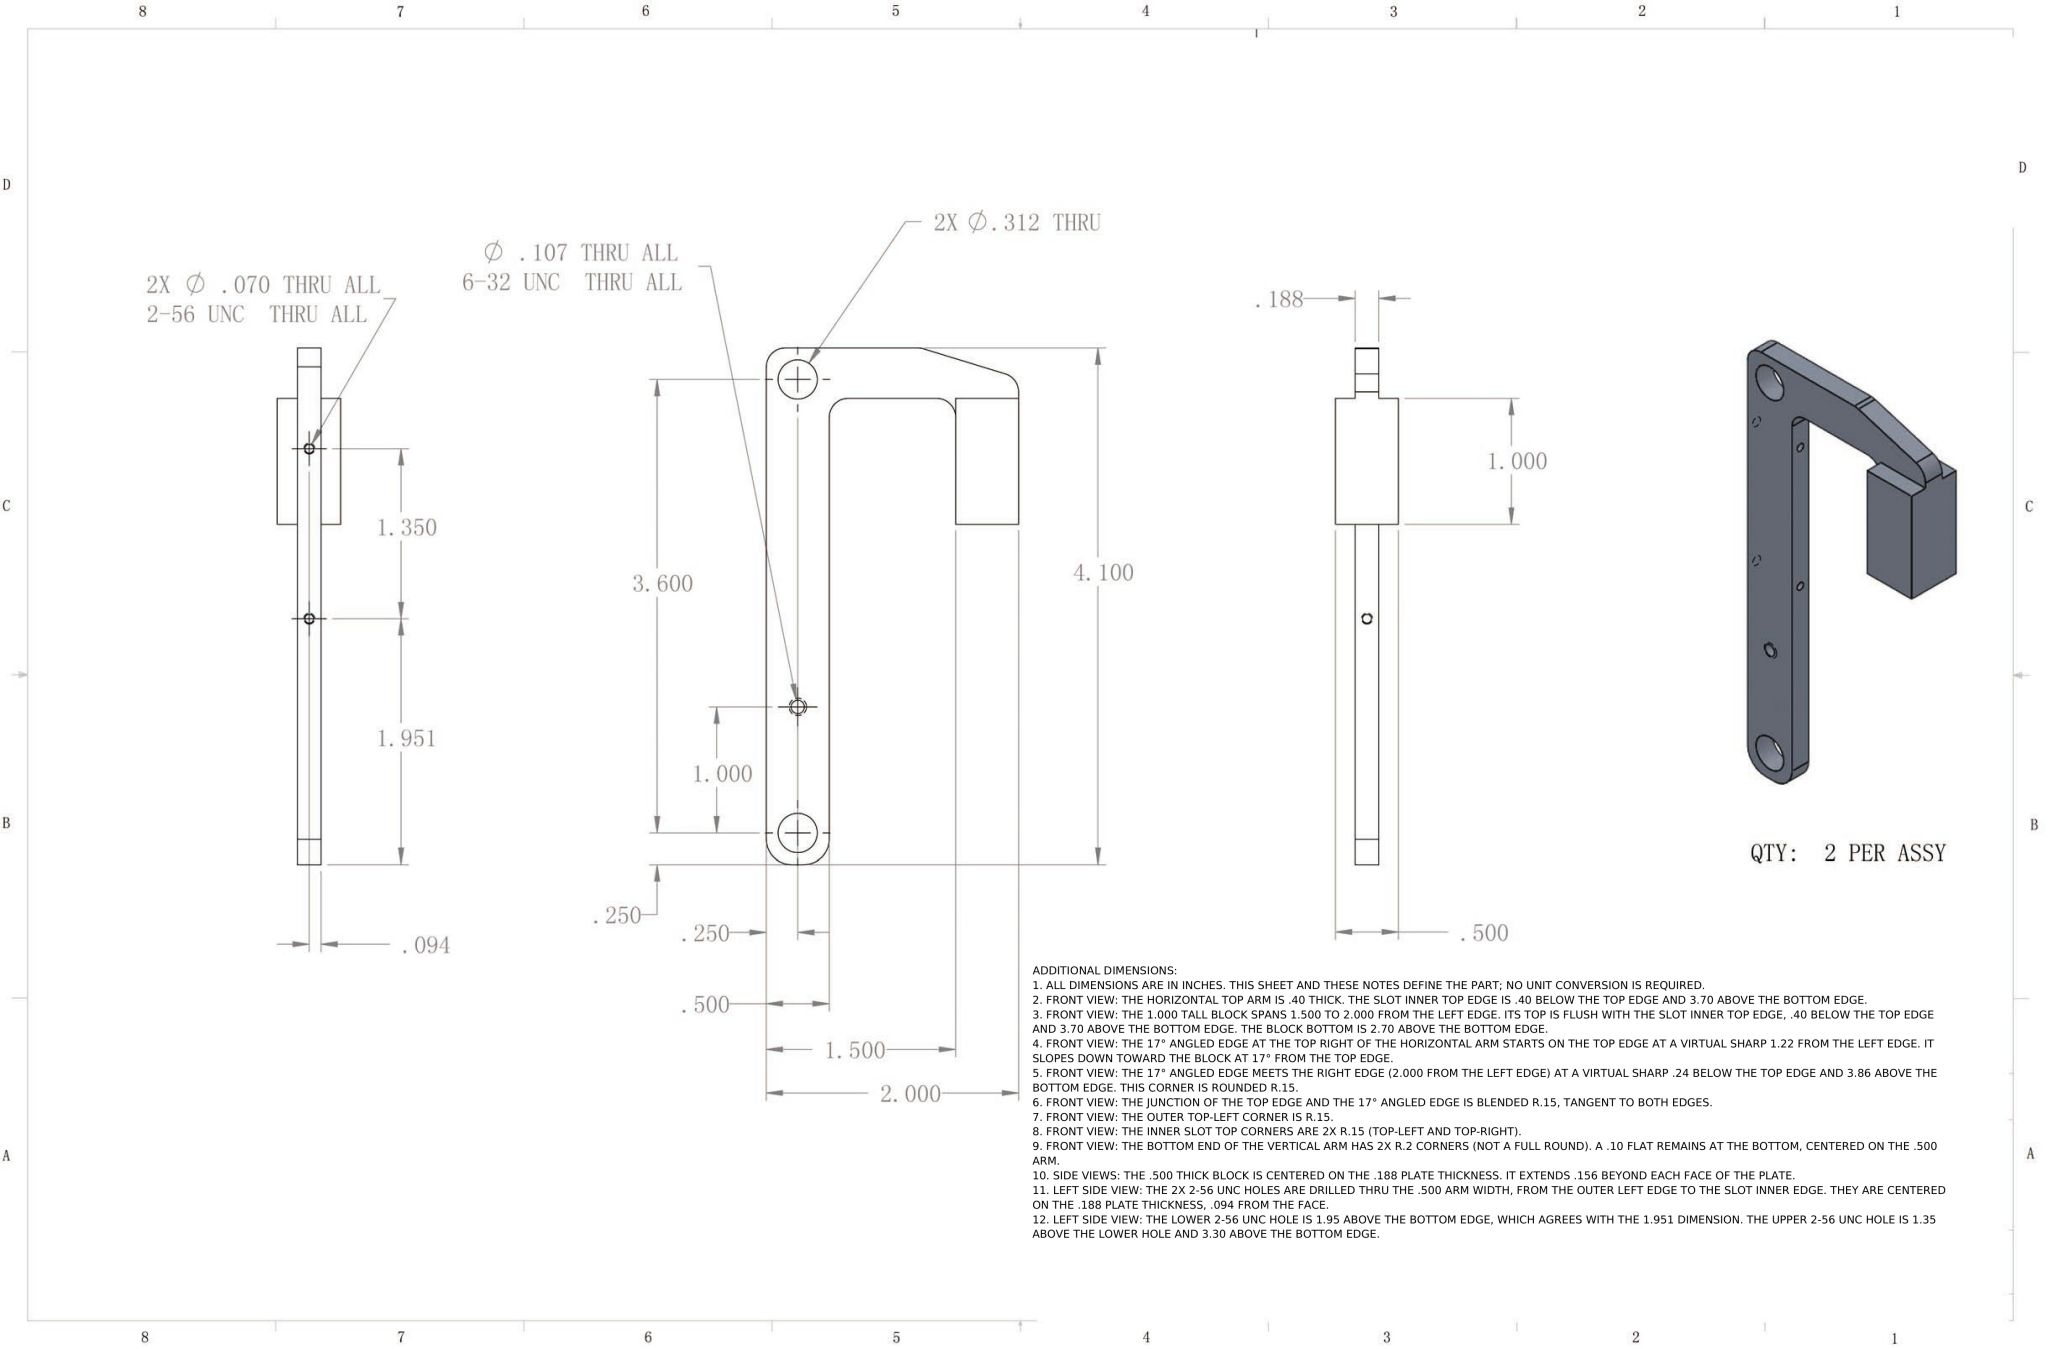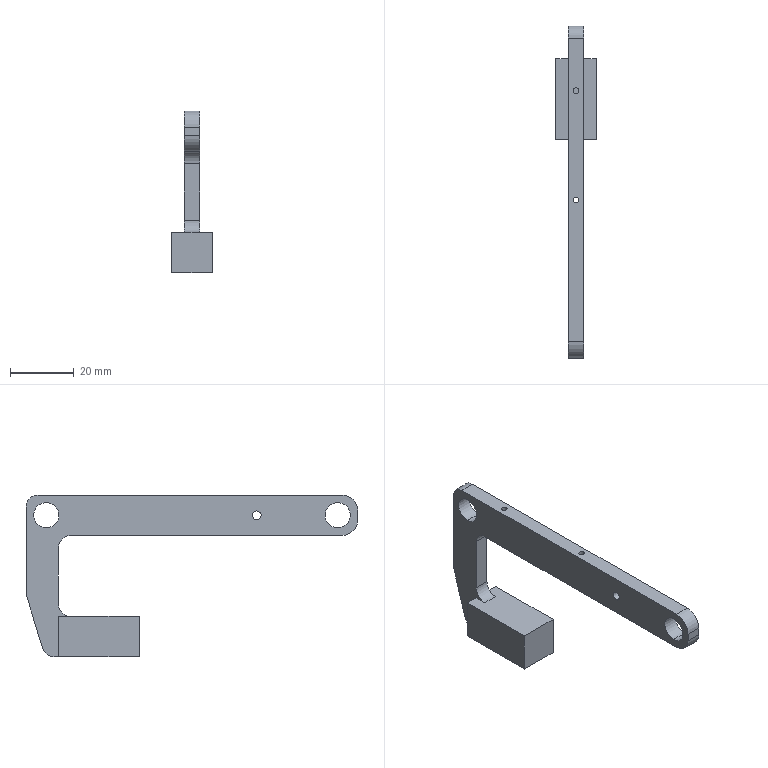Part | NX | drawing in inches | 1 solid | 32 faces | box 12.7 x 104.14 x 50.8 mm | volume 11350 mm3 | cylinder 17 | plane 15 | commonest cylinder face diameters 7.62 x5 1.778 x4 7.925 x4 2.705 x2 10.16 x2